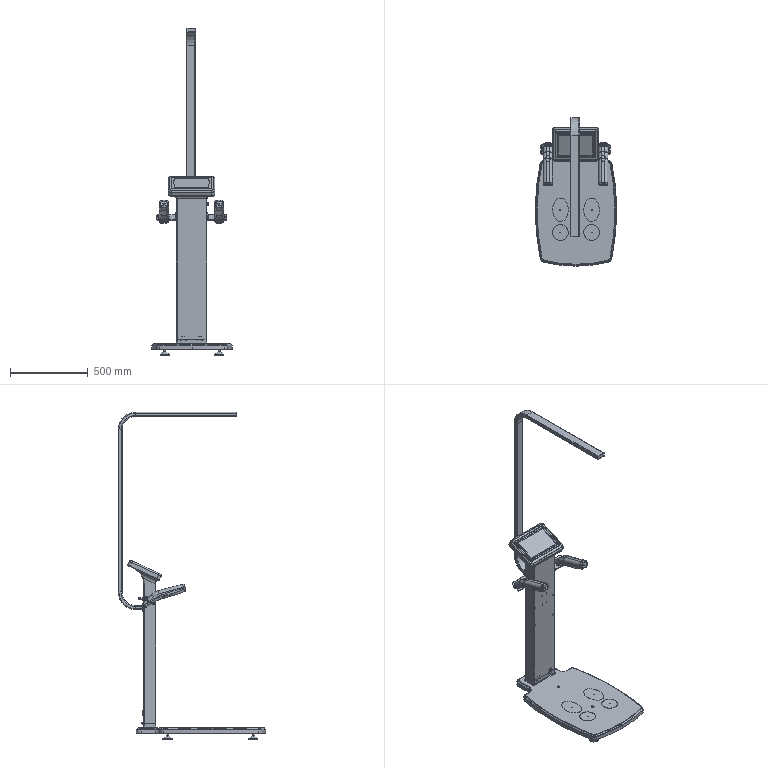Assembly | SolidWorks | mm | 47 component files | 54 solids | 2574 faces | box 521.26 x 947.82 x 2100 mm | volume 8261923 mm3 | plane 1176 | cylinder 875 | torus 188 | spline 175 | cone 146 | sphere 14 | commonest cylinder face diameters 5 x104 2 x102 10 x88 1 x46 6 x43 2.5 x38 20 x36 3 x32
Bill of materials:
10.1InchMotherboard | 1 |  | Thin, nearly square flat plate with small rounded corners. A row of protruding blocks of different sizes runs along one edge, and several of them have recesses, slots or round openings.
10.1InchScreen | 1 |  | Thin rectangular plate with small corner radii. The edge views show a slight step or offset near both short ends.
AviationExternalConnector | 2 |  | Stepped body of revolution. It has a large flanged end with a recessed face, a cylindrical barrel, a short conical step-down, a hexagonal section and a smaller cylindrical end.
AviationPlug | 2 |  | Solid cylinder with a single narrow raised collar placed off-center along its length.
BA850-01-02-01New | 2 | AISI 304 | Thin flat circular disc of uniform thickness.
BA850-01-03-01New | 2 | AISI 304 | Thin flat disc that appears to have an elliptical outline, with uniform thickness.
BaseBottomPlate | 1 |  | Thin flat plate with a barrel-shaped outline (convex curved long sides) and a narrower rectangular tab at one end, joined by filleted inside corners.
BaseTopCover | 1 |  | Thicker plate with the same barrel-shaped outline and end tab. It has rounded edges, and the tab carries a raised hollow rectangular frame.
BodyCompositionBoard | 1 |  | Flat rectangular plate of uniform thickness with four through holes, one near each corner.
Column | 1 |  | Long post with a rectangular cross-section. At the top is an angled rectangular head with a rounded rim and a tapered, open cavity.
ColumnCover | 1 |  | Tall, narrow, thin rectangular sheet with small holes spaced along both long edges.
FootPad | 4 | Stainless Steel (Ferritic) | Solid body of revolution: a short cylindrical disc base topped by a conical section that narrows into a slender cylindrical stem.
GB-T15389-1994-M3-20StudNew | 4 |  | Solid straight cylindrical pin with one flat end and one chamfered end.
GQ16F_10 | 1 |  | Cylindrical body with a flanged front bezel that has a chamfered rim, a flat circular face inset slightly inside the rim, a hexagonal nut-like ring part-way along the cylindrical barrel, a stepped rear collar, and two parallel flat rear tabs. Each tab has a round through-hole and a short cylindrical tip, and a thin central blade sits between the two tabs. The overall form looks like a panel-mount pushbutton-style component.
HandleBracket | 2 |  | Flat L-shaped bracket plate. One end has a short perpendicular flange. The plate has a large rounded-rectangular cutout that opens to the far end through a narrow slot, giving a C-shaped clip outline.
HeightMeasurement | 1 |  | Thin flat strip bent into a hook-like profile. It has a long straight leg, a radiused 90-degree bend to a second straight leg, and a short radiused return at the other end.
HeightSensor | 1 |  | Thin square plate with a shallow round boss on one face. The boss has a rounded edge.
Hinge1 | 3 |  | Flat leaf plate with two rolled knuckles, one at each end of one edge, and a rectangular recess between them. The plate has two round through-holes.
Hinge2 | 3 |  | Rectangular flat leaf plate with one continuous rolled knuckle along one edge and two round through-holes.
HandleLowerElectrode | 2 | Stainless Steel (Ferritic) | Thin curved shell with an oval outline. It has a gently curved base surface and two upright wall segments rising from its sides, giving a U-shaped front profile.
HandleLowerPart | 2 |  | Long, open, tray-like shell with a rounded-rectangular outline and thin walls, curved along its length. It has a large elliptical opening in the floor and small notches in the rim at both ends.
HandleUpperElectrode | 2 | Stainless Steel (Ferritic) | Thin oval disc of constant thickness, slightly bent along its long axis.
HandleUpperPart | 2 |  | Long, curved, hollow cover shell with rounded ends and a convex outer surface. It has an oval through-hole near one end and small notches at the end edges.
Level | 1 |  | Short cylindrical disc or cap with a filleted top edge and a recessed cross-shaped (X) groove in the top face.
Three-in-oneSocket-ScrewFasteningType | 1 |  | Box-shaped body with a flange plate shaped like an elongated hexagon, with two mounting holes. Flat blade-style tabs and small pin-like leads stick out of the back. A sloped feature extends past the flange on the front side.
USBSocket | 2 |  | Flanged body that tapers from a wide end to a narrow end. The wide end has a flat mounting flange with rounded ends and one small through-hole near each end. The body has rounded edges and narrows to a stepped cylindrical boss, with a longer, thinner cylindrical rod sticking out of the boss.
WeightSensor100KgNew | 1 |  | Rectangular bar-shaped block. Each end has a raised pad with three small round holes in a triangular pattern. The middle section is slightly recessed on the top and bottom faces. A transverse through-opening runs through the middle, shaped like two round holes joined by a narrow slot (dog-bone). A small cylindrical stub sticks out of one end face.
Mates:
1. coincident | BaseTopCover-1 face at (965.186, 1488.312, 1401.454) dir (0, 0, -1) | BaseBottomPlate-1 face at (1140.186, 1208.312, 1401.454) dir (0, 0, -1)
2. parallel | BaseBottomPlate-1 face at (1001.186, 1488.312, 1406.455) dir (-1, 0, 0) | BaseTopCover-1 face at (995.186, 1488.312, 1401.454) dir (-1, 0, 0)
3. parallel | BaseBottomPlate-1 face at (1025.186, 1602.312, 1406.455) dir (0, 1, 0) | BaseTopCover-1 face at (1250.186, 1608.312, 1401.454) dir (0, 1, 0)
4. coincident | BaseTopCover-1 face at (1040.186, 1488.312, 1466.454) dir (-1, 0, 0) | Column-1 face at (1040.186, 1563.312, 2632.705) dir (-1, 0, 0)
5. distance | BaseBottomPlate-1 face at (1140.186, 1208.312, 1406.454) dir (0, 0, 1) | BA850-01-02-01New-1 face at (1240.186, 993.812, 1434.454) dir (0, 0, -1)
6. concentric | BA850-01-02-01New-1 face at (1240.186, 993.812, 1434.454) dir (0, 0, 1) r 50 | GB-T15389-1994-M3-20StudNew-1 face at (1240.186, 993.812, 1419.454) dir (0, 0, 1) r 1.5
7. coincident | BA850-01-02-01New-1 face at (1240.186, 993.812, 1434.454) dir (0, 0, -1) | GB-T15389-1994-M3-20StudNew-1 face at (1240.186, 993.812, 1434.454) dir (0, 0, 1)
8. coincident | BA850-01-02-01New-1 face at (1240.186, 993.812, 1436.454) dir (0, 0, 1) | BA850-01-03-01New-1 face at (1240.186, 1138.812, 1436.454) dir (0, 0, 1)
9. distance | BA850-01-03-01New-1 plane at (1240.186, 1138.812, 1434.454) dir (0, -1, 0) | BA850-01-02-01New-1 face at (1240.186, 993.812, 1434.454) dir (0, 0, 1) r 50
10. coincident | GB-T15389-1994-M3-20StudNew-1 face at (1240.186, 993.812, 1419.454) dir (0, 0, -1) | GB-T15389-1994-M3-20StudNew-5 face at (1240.186, 1138.812, 1419.454) dir (0, 0, -1)
11. concentric | BaseBottomPlate-1 face at (1315.186, 858.312, 1401.453) dir (0, 0, 1) r 6.25 | FootPad-1 face at (1315.186, 858.312, 1361.454) dir (0, 0, -1) r 6
12. distance | FootPad-1 face at (1345.186, 858.312, 1361.454) dir (0, 0, -1) | BaseBottomPlate-1 face at (1140.186, 1208.312, 1401.454) dir (0, 0, -1)
13. coincident | Column-1 face at (1217.686, 1497.312, 1900.983) dir (0, 1, 0) | 10.1InchMotherboard-1 face at (1220.486, 1497.312, 2063.133) dir (0, -1, 0)
14. concentric | Column-1 face at (1057.686, 1497.312, 1900.983) dir (0, -1, 0) r 1.25 | 10.1InchMotherboard-1 face at (1057.686, 1497.312, 1900.983) dir (0, 1, 0) r 1.95
15. parallel | Column-1 face at (1044.186, 1563.312, 2632.705) dir (1, 0, 0) | 10.1InchMotherboard-1 face at (1053.486, 1498.912, 2063.133) dir (-1, 0, 0)
16. coincident | Column-1 face at (987.686, 1446.407, 2419.312) dir (0, -0.4226, 0.9063) | 10.1InchScreen-1 face at (1262.686, 1474.956, 2432.624) dir (0, -0.4226, 0.9063)
17. coincident | Column-1 face at (1266.186, 1630.991, 2502.626) dir (-1, 0, 0) | 10.1InchScreen-1 face at (1266.186, 1474.956, 2432.624) dir (1, 0, 0)
18. coincident | Column-1 face at (1009.186, 1630.991, 2502.626) dir (0, -0.9063, -0.4226) | 10.1InchScreen-1 face at (1013.136, 1629.935, 2504.892) dir (0, 0.9063, 0.4226)
19. coincident | Column-1 face at (1160.186, 1492.312, 2028.683) dir (0, 1, 0) | BodyCompositionBoard-2 face at (1141.186, 1492.312, 2062.333) dir (0, -1, 0)
20. concentric | Column-1 face at (1122.186, 1492.312, 2028.683) dir (0, -1, 0) r 1.5 | BodyCompositionBoard-2 face at (1122.186, 1492.312, 2028.683) dir (0, 1, 0) r 1.5
21. concentric | Column-1 face at (1160.186, 1492.312, 2095.983) dir (0, -1, 0) r 1.5 | BodyCompositionBoard-2 face at (1160.186, 1492.312, 2095.983) dir (0, 1, 0) r 1.5
22. coincident | Column-1 face at (1040.186, 1563.312, 2632.705) dir (0, 1, 0) | ColumnCover-1 face at (1137.686, 1563.312, 1865.983) dir (0, 1, 0)
23. concentric | Column-1 face at (1065.186, 1559.312, 2143.483) dir (0, 1, 0) r 1.25 | ColumnCover-1 face at (1065.186, 1563.312, 2143.483) dir (0, 1, 0) r 1.7
24. concentric | Column-1 face at (1210.186, 1559.312, 1588.483) dir (0, 1, 0) r 1.25 | ColumnCover-1 face at (1210.186, 1563.312, 1588.483) dir (0, 1, 0) r 1.7
25. coincident | Column-1 face at (1235.186, 1563.312, 2632.705) dir (1, 0, 0) | GQ16F_10-1 face at (1235.186, 1512.412, 2335.983) dir (-1, 0, 0)
26. concentric | Column-1 face at (1230.186, 1523.312, 2335.983) dir (1, 0, 0) r 8 | GQ16F_10-1 face at (1287.814, 1523.312, 2335.983) dir (1, 0, 0) r 8
27. concentric | Column-1 face at (1197.686, 1449.696, 2265.983) dir (0, 1, 0) r 7.5 | AviationPlug-1 face at (1197.686, 1570.312, 2265.983) dir (0, -1, 0) r 7.5
28. coincident | Column-1 face at (1040.186, 1563.312, 2632.705) dir (0, 1, 0) | AviationPlug-1 face at (1197.686, 1563.312, 2265.983) dir (0, -1, 0)
29. coincident | Column-1 face at (1040.186, 1563.312, 2632.705) dir (0, 1, 0) | Three-in-oneSocket-ScrewFasteningType-1 face at (1056.148, 1563.312, 1532.383) dir (0, -1, 0)
30. coincident | Column-1 face at (1107.186, 1559.312, 1518.783) dir (0, 0, 1) | Three-in-oneSocket-ScrewFasteningType-1 face at (1099.736, 1546.112, 1518.783) dir (0, 0, -1)
31. coincident | Column-1 face at (1060.186, 1559.312, 1545.983) dir (1, 0, 0) | Three-in-oneSocket-ScrewFasteningType-1 face at (1060.186, 1546.112, 1520.083) dir (-1, 0, 0)
32. concentric | Column-1 face at (1134.186, 1558.312, 1522.483) dir (0, 1, 0) r 1.5 | USBSocket-1 face at (1134.186, 1559.312, 1522.483) dir (0, 1, 0) r 1.25
33. concentric | USBSocket-1 face at (1163.186, 1559.312, 1522.483) dir (0, 1, 0) r 1.25 | Column-1 face at (1163.186, 1558.312, 1522.483) dir (0, 1, 0) r 1.5
34. coincident | Column-1 edge at (1142.186, 1559.312, 1518.983) dir (1, 0, 0) | USBSocket-1 face at (1156.686, 1559.312, 1528.483) dir (0, 1, 0)
35. concentric | AviationPlug-1 face at (1197.686, 1570.312, 2265.983) dir (0, -1, 0) r 7.5 | AviationExternalConnector-1 face at (1197.686, 1596.512, 2265.983) dir (0, 1, 0) r 8.7
36. coincident | AviationPlug-1 face at (1197.686, 1565.312, 2265.983) dir (0, 1, 0) | AviationExternalConnector-1 edge at (1197.686, 1565.312, 2265.983) dir (0, 1, 0) r 8.7
37. coincident | BaseTopCover-1 face at (1045.186, 1563.312, 1466.454) dir (0, 1, 0) | Column-1 face at (1040.186, 1563.312, 2632.705) dir (0, 1, 0)
38. coincident | BaseTopCover-1 face at (1045.186, 1488.312, 1466.454) dir (0, 0, 1) | Column-1 face at (1040.186, 1483.312, 1466.454) dir (0, 0, -1)
39. coincident | BaseTopCover-1 face at (1229.186, 1488.312, 1466.454) dir (0, 1, 0) | Hinge-1/Hinge1-1 face at (1215.186, 1488.312, 1451.454) dir (0, -1, 0)
40. distance | Hinge-1/Hinge1-1 face at (1215.186, 1493.312, 1471.454) dir (-1, 0, 0) r 3 | BaseTopCover-1 face at (1045.186, 1488.312, 1466.454) dir (0, 0, 1)
41. distance | Hinge-1/Hinge1-1 face at (1215.186, 1490.312, 1471.454) dir (1, 0, 0) | BaseTopCover-1 face at (1235.186, 1558.312, 1466.454) dir (1, 0, 0)
42. concentric | BaseTopCover-1 face at (1140.186, 1358.312, 1433.454) dir (0, 0, 1) r 7.5 | Level-1 face at (1140.186, 1358.312, 1433.454) dir (0, 0, 1) r 7.5
43. distance | Level-1 face at (1140.186, 1358.312, 1438.454) dir (0, 0, 1) | BaseTopCover-1 face at (965.186, 1488.312, 1436.454) dir (0, 0, 1)
44. coincident | Column-1 face at (1040.186, 1563.312, 2632.705) dir (0, 1, 0) | Hinge-3/Hinge1-1 face at (1112.106, 1563.312, 1486.454) dir (0, -1, 0)
45. coincident | Column-1 edge at (1230.186, 1563.312, 1466.454) dir (-1, 0, 0) | Hinge-3/Hinge1-1 edge at (1152.106, 1563.312, 1466.454) dir (1, 0, 0)
46. coincident | Column-1 face at (1040.186, 1563.312, 2632.705) dir (0, 1, 0) | HeightMeasurement-1 face at (1107.686, 1563.312, 2216.454) dir (0, -1, 0)
47. distance | Column-1 face at (1235.186, 1563.312, 2632.705) dir (1, 0, 0) | HeightMeasurement-1 face at (1177.686, 1568.312, 2216.454) dir (1, 0, 0)
48. distance | BaseTopCover-1 face at (965.186, 1488.312, 1436.454) dir (0, 0, 1) | HeightMeasurement-1 face at (1107.686, 963.312, 3436.454) dir (0, 0, -1)
49. coincident | HeightMeasurement-1 edge at (1132.686, 1063.312, 3438.454) dir (0, 0, -1) r 19.2 | HeightSensor-1 face at (1132.686, 1063.312, 3438.454) dir (0, 0, -1)
50. concentric | HeightMeasurement-1 face at (1132.686, 1063.312, 3461.455) dir (0, 0, -1) r 19.2 | HeightSensor-1 face at (1132.686, 1063.312, 3433.454) dir (0, 0, 1) r 19.2
51. coincident | Column-1 face at (1235.186, 1563.312, 2632.705) dir (1, 0, 0) | HandleBracket-1 face at (1235.186, 1484.652, 2249.599) dir (-1, 0, 0)
52. distance | Column-1 face at (1040.186, 1483.312, 2632.705) dir (0, -1, 0) | HandleBracket-1 face at (1235.186, 1498.312, 2245.939) dir (1, 0, 0) r 2.5
53. angle | HumanHandle-1/UpperHandle-1/HandleUpperPart-1 face at (1345.186, 1492.734, 2310.127) dir (0, 0.7071, 0.7071) | HandleBracket-1 face at (1240.186, 1494.652, 2232.278) dir (0, -0.5, 0.866)
54. angle | HandleBracket-1 face at (1240.186, 1494.652, 2232.278) dir (0, -0.5, 0.866) | Column-1 face at (1040.186, 1483.312, 2632.705) dir (0, -1, 0)
55. distance | HumanHandle-1/UpperHandle-1/HandleUpperPart-1 face at (1285.186, 1287.809, 2302.92) dir (-1, 0, 0) | HandleBracket-1 face at (1282.686, 1525.788, 2273.349) dir (1, 0, 0)
56. coincident | Column-1 face at (1040.186, 1563.312, 2632.705) dir (-1, 0, 0) | HandleBracket-3 face at (1040.186, 1545.273, 2284.599) dir (1, 0, 0)
57. distance | Column-1 face at (1040.186, 1483.312, 2632.705) dir (0, -1, 0) | HandleBracket-3 face at (1040.186, 1498.312, 2245.939) dir (-1, 0, 0) r 2.5
58. coincident | HandleBracket-1 face at (1240.186, 1494.652, 2232.278) dir (0, -0.5, 0.866) | HandleBracket-3 face at (1035.186, 1555.273, 2267.278) dir (0, -0.5, 0.866)
59. concentric | Hinge1-1 face at (1030.925, 1016.752, 1027.323) dir (-1, 0, 0) r 3 | Hinge2-2 face at (990.925, 1016.752, 1027.323) dir (1, 0, 0) r 3
60. coincident | Hinge1-1 face at (1020.925, 1022.752, 1022.323) dir (-1, 0, 0) | Hinge2-2 face at (1020.925, 1016.752, 1027.323) dir (1, 0, 0)
61. coincident | Hinge1-1 face at (1030.925, 996.752, 1032.323) dir (0, 0, 1) | Hinge2-2 face at (990.925, 1036.752, 1032.323) dir (0, 0, 1)
62. coincident | UpperHandle-1/HandleUpperPart-1 plane at (-23.603, -115.589, 556.816) dir (1, 0, 0) | LowerHandle-1/HandleLowerPart-1 plane at (-23.603, -115.589, 556.816) dir (1, 0, 0)
63. coincident | UpperHandle-1/HandleUpperPart-1 plane at (-23.603, -115.589, 556.816) dir (0, -1, 0) | LowerHandle-1/HandleLowerPart-1 plane at (-23.603, -115.589, 556.816) dir (0, -1, 0)
64. coincident | UpperHandle-1/HandleUpperPart-1 plane at (-23.603, -115.589, 556.816) dir (0, 0, 1) | LowerHandle-1/HandleLowerPart-1 plane at (-23.603, -115.589, 556.816) dir (0, 0, 1)
65. coincident | HandleLowerPart-1 plane at (-40.809, -160.062, 280.523) dir (0, -1, 0) | HandleLowerElectrode-1 plane at (-40.809, -160.062, 280.523) dir (0, -1, 0)
66. coincident | HandleLowerPart-1 plane at (-40.809, -160.062, 280.523) dir (0, 0, 1) | HandleLowerElectrode-1 plane at (-40.809, -160.062, 280.523) dir (0, 0, 1)
67. coincident | HandleLowerPart-1 plane at (-40.809, -160.062, 280.523) dir (1, 0, 0) | HandleLowerElectrode-1 plane at (-40.809, -160.062, 280.523) dir (1, 0, 0)
68. coincident | HandleUpperPart-1 plane at (-24.538, -159.88, 266.195) dir (0, -1, 0) | HandleUpperElectrode-1 plane at (-24.538, -159.88, 266.195) dir (0, -1, 0)
69. coincident | HandleUpperPart-1 plane at (-24.538, -159.88, 266.195) dir (0, 0, 1) | HandleUpperElectrode-1 plane at (-24.538, -159.88, 266.195) dir (0, 0, 1)
70. coincident | HandleUpperPart-1 plane at (-24.538, -159.88, 266.195) dir (1, 0, 0) | HandleUpperElectrode-1 plane at (-24.538, -159.88, 266.195) dir (1, 0, 0)